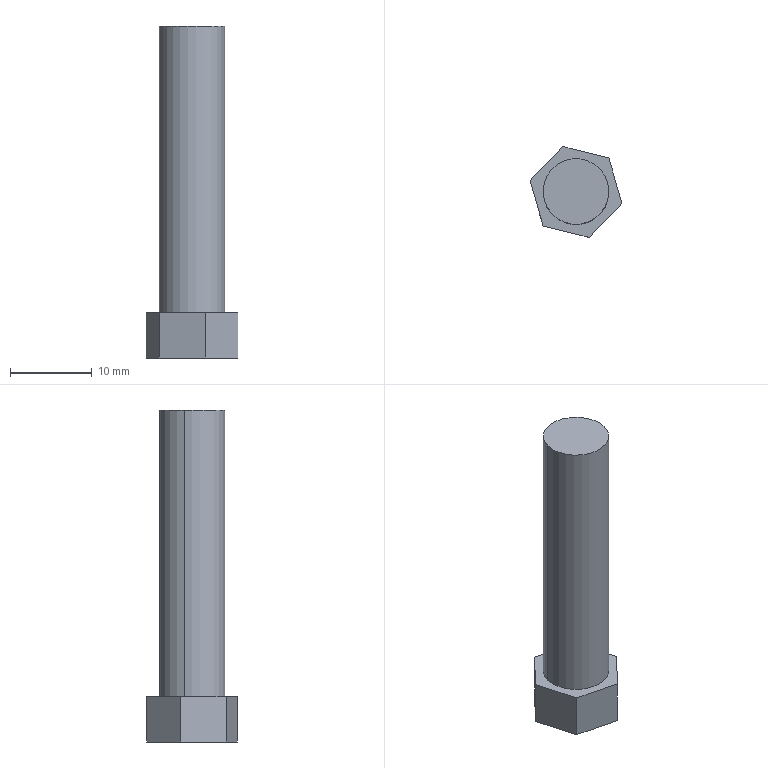Component | SolidWorks | 8Bolt35-1 | 1 solid | 11 faces | box 11.21 x 11.09 x 40.5 mm | volume 2236 mm3 | plane 9 | cylinder 2 | commonest cylinder face diameters 8 x2
STEP:
#1=COLOUR_RGB('',0.7922,0.8196,0.9333);
#2=FILL_AREA_STYLE_COLOUR('',#1);
#3=FILL_AREA_STYLE('',(#2));
#4=SURFACE_STYLE_FILL_AREA(#3);
#5=SURFACE_SIDE_STYLE('',(#4));
#6=SURFACE_STYLE_USAGE(.BOTH.,#5);
#7=PRESENTATION_STYLE_ASSIGNMENT((#6));
#8=CARTESIAN_POINT('',(3.878,5.256,2.511));
#9=VERTEX_POINT('',#8);
#10=CARTESIAN_POINT('',(3.572,5.332,2.511));
#11=VERTEX_POINT('',#10);
#12=CARTESIAN_POINT('',(3.725,5.294,2.511));
#13=DIRECTION('',(0.,0.,1.));
#14=DIRECTION('',(0.9707,-0.2403,0.));
#15=AXIS2_PLACEMENT_3D('',#12,#13,#14);
#16=CIRCLE('',#15,0.1575);
#17=EDGE_CURVE('',#9,#11,#16,.T.);
#18=ORIENTED_EDGE('',*,*,#17,.F.);
#19=CARTESIAN_POINT('',(3.878,5.256,1.133));
#20=VERTEX_POINT('',#19);
#21=CARTESIAN_POINT('',(3.878,5.256,2.511));
#22=DIRECTION('',(0.,0.,-1.));
#23=VECTOR('',#22,39.37);
#24=LINE('',#21,#23);
#25=EDGE_CURVE('',#9,#20,#24,.T.);
#26=ORIENTED_EDGE('',*,*,#25,.T.);
#27=CARTESIAN_POINT('',(3.572,5.332,1.133));
#28=VERTEX_POINT('',#27);
#29=CARTESIAN_POINT('',(3.725,5.294,1.133));
#30=DIRECTION('',(0.,0.,1.));
#31=DIRECTION('',(0.9707,-0.2403,0.));
#32=AXIS2_PLACEMENT_3D('',#29,#30,#31);
#33=CIRCLE('',#32,0.1575);
#34=EDGE_CURVE('',#20,#28,#33,.T.);
#35=ORIENTED_EDGE('',*,*,#34,.T.);
#36=CARTESIAN_POINT('',(3.572,5.332,2.511));
#37=DIRECTION('',(0.,0.,-1.));
#38=VECTOR('',#37,39.37);
#39=LINE('',#36,#38);
#40=EDGE_CURVE('',#11,#28,#39,.T.);
#41=ORIENTED_EDGE('',*,*,#40,.F.);
#42=EDGE_LOOP('',(#18,#26,#35,#41));
#43=FACE_OUTER_BOUND('',#42,.T.);
#44=CARTESIAN_POINT('',(3.725,5.294,2.511));
#45=DIRECTION('',(0.,0.,-1.));
#46=DIRECTION('',(-0.9707,0.2403,0.));
#47=AXIS2_PLACEMENT_3D('',#44,#45,#46);
#48=CYLINDRICAL_SURFACE('',#47,0.1575);
#49=ADVANCED_FACE('',(#43),#48,.T.);
#50=CARTESIAN_POINT('',(3.788,5.075,0.9168));
#51=VERTEX_POINT('',#50);
#52=CARTESIAN_POINT('',(3.946,5.239,0.9168));
#53=VERTEX_POINT('',#52);
#54=CARTESIAN_POINT('',(3.788,5.075,0.9168));
#55=DIRECTION('',(0.6935,0.7205,0.));
#56=VECTOR('',#55,39.37);
#57=LINE('',#54,#56);
#58=EDGE_CURVE('',#51,#53,#57,.T.);
#59=ORIENTED_EDGE('',*,*,#58,.T.);
#60=CARTESIAN_POINT('',(3.946,5.239,1.133));
#61=VERTEX_POINT('',#60);
#62=CARTESIAN_POINT('',(3.946,5.239,1.133));
#63=DIRECTION('',(0.,0.,-1.));
#64=VECTOR('',#63,39.37);
#65=LINE('',#62,#64);
#66=EDGE_CURVE('',#61,#53,#65,.T.);
#67=ORIENTED_EDGE('',*,*,#66,.F.);
#68=CARTESIAN_POINT('',(3.788,5.075,1.133));
#69=VERTEX_POINT('',#68);
#70=CARTESIAN_POINT('',(3.788,5.075,1.133));
#71=DIRECTION('',(0.6935,0.7205,0.));
#72=VECTOR('',#71,39.37);
#73=LINE('',#70,#72);
#74=EDGE_CURVE('',#69,#61,#73,.T.);
#75=ORIENTED_EDGE('',*,*,#74,.F.);
#76=CARTESIAN_POINT('',(3.788,5.075,1.133));
#77=DIRECTION('',(0.,0.,-1.));
#78=VECTOR('',#77,39.37);
#79=LINE('',#76,#78);
#80=EDGE_CURVE('',#69,#51,#79,.T.);
#81=ORIENTED_EDGE('',*,*,#80,.T.);
#82=EDGE_LOOP('',(#59,#67,#75,#81));
#83=FACE_OUTER_BOUND('',#82,.T.);
#84=CARTESIAN_POINT('',(3.788,5.075,1.133));
#85=DIRECTION('',(-0.7205,0.6935,0.));
#86=DIRECTION('',(-0.6935,-0.7205,0.));
#87=AXIS2_PLACEMENT_3D('',#84,#85,#86);
#88=PLANE('',#87);
#89=ADVANCED_FACE('',(#83),#88,.F.);
#90=CARTESIAN_POINT('',(3.883,5.458,0.9168));
#91=VERTEX_POINT('',#90);
#92=CARTESIAN_POINT('',(3.946,5.239,0.9168));
#93=DIRECTION('',(-0.2772,0.9608,0.));
#94=VECTOR('',#93,39.37);
#95=LINE('',#92,#94);
#96=EDGE_CURVE('',#53,#91,#95,.T.);
#97=ORIENTED_EDGE('',*,*,#96,.T.);
#98=CARTESIAN_POINT('',(3.883,5.458,1.133));
#99=VERTEX_POINT('',#98);
#100=CARTESIAN_POINT('',(3.883,5.458,1.133));
#101=DIRECTION('',(0.,0.,-1.));
#102=VECTOR('',#101,39.37);
#103=LINE('',#100,#102);
#104=EDGE_CURVE('',#99,#91,#103,.T.);
#105=ORIENTED_EDGE('',*,*,#104,.F.);
#106=CARTESIAN_POINT('',(3.946,5.239,1.133));
#107=DIRECTION('',(-0.2772,0.9608,0.));
#108=VECTOR('',#107,39.37);
#109=LINE('',#106,#108);
#110=EDGE_CURVE('',#61,#99,#109,.T.);
#111=ORIENTED_EDGE('',*,*,#110,.F.);
#112=ORIENTED_EDGE('',*,*,#66,.T.);
#113=EDGE_LOOP('',(#97,#105,#111,#112));
#114=FACE_OUTER_BOUND('',#113,.T.);
#115=CARTESIAN_POINT('',(3.946,5.239,1.133));
#116=DIRECTION('',(-0.9608,-0.2772,0.));
#117=DIRECTION('',(0.2772,-0.9608,0.));
#118=AXIS2_PLACEMENT_3D('',#115,#116,#117);
#119=PLANE('',#118);
#120=ADVANCED_FACE('',(#114),#119,.F.);
#121=CARTESIAN_POINT('',(3.662,5.512,0.9168));
#122=VERTEX_POINT('',#121);
#123=CARTESIAN_POINT('',(3.883,5.458,0.9168));
#124=DIRECTION('',(-0.9707,0.2403,0.));
#125=VECTOR('',#124,39.37);
#126=LINE('',#123,#125);
#127=EDGE_CURVE('',#91,#122,#126,.T.);
#128=ORIENTED_EDGE('',*,*,#127,.T.);
#129=CARTESIAN_POINT('',(3.662,5.512,1.133));
#130=VERTEX_POINT('',#129);
#131=CARTESIAN_POINT('',(3.662,5.512,1.133));
#132=DIRECTION('',(0.,0.,-1.));
#133=VECTOR('',#132,39.37);
#134=LINE('',#131,#133);
#135=EDGE_CURVE('',#130,#122,#134,.T.);
#136=ORIENTED_EDGE('',*,*,#135,.F.);
#137=CARTESIAN_POINT('',(3.883,5.458,1.133));
#138=DIRECTION('',(-0.9707,0.2403,0.));
#139=VECTOR('',#138,39.37);
#140=LINE('',#137,#139);
#141=EDGE_CURVE('',#99,#130,#140,.T.);
#142=ORIENTED_EDGE('',*,*,#141,.F.);
#143=ORIENTED_EDGE('',*,*,#104,.T.);
#144=EDGE_LOOP('',(#128,#136,#142,#143));
#145=FACE_OUTER_BOUND('',#144,.T.);
#146=CARTESIAN_POINT('',(3.883,5.458,1.133));
#147=DIRECTION('',(-0.2403,-0.9707,0.));
#148=DIRECTION('',(0.,0.,-1.));
#149=AXIS2_PLACEMENT_3D('',#146,#147,#148);
#150=PLANE('',#149);
#151=ADVANCED_FACE('',(#145),#150,.F.);
#152=CARTESIAN_POINT('',(3.504,5.348,0.9168));
#153=VERTEX_POINT('',#152);
#154=CARTESIAN_POINT('',(3.662,5.512,0.9168));
#155=DIRECTION('',(-0.6935,-0.7205,0.));
#156=VECTOR('',#155,39.37);
#157=LINE('',#154,#156);
#158=EDGE_CURVE('',#122,#153,#157,.T.);
#159=ORIENTED_EDGE('',*,*,#158,.T.);
#160=CARTESIAN_POINT('',(3.504,5.348,1.133));
#161=VERTEX_POINT('',#160);
#162=CARTESIAN_POINT('',(3.504,5.348,1.133));
#163=DIRECTION('',(0.,0.,-1.));
#164=VECTOR('',#163,39.37);
#165=LINE('',#162,#164);
#166=EDGE_CURVE('',#161,#153,#165,.T.);
#167=ORIENTED_EDGE('',*,*,#166,.F.);
#168=CARTESIAN_POINT('',(3.662,5.512,1.133));
#169=DIRECTION('',(-0.6935,-0.7205,0.));
#170=VECTOR('',#169,39.37);
#171=LINE('',#168,#170);
#172=EDGE_CURVE('',#130,#161,#171,.T.);
#173=ORIENTED_EDGE('',*,*,#172,.F.);
#174=ORIENTED_EDGE('',*,*,#135,.T.);
#175=EDGE_LOOP('',(#159,#167,#173,#174));
#176=FACE_OUTER_BOUND('',#175,.T.);
#177=CARTESIAN_POINT('',(3.662,5.512,1.133));
#178=DIRECTION('',(0.7205,-0.6935,0.));
#179=DIRECTION('',(0.6935,0.7205,0.));
#180=AXIS2_PLACEMENT_3D('',#177,#178,#179);
#181=PLANE('',#180);
#182=ADVANCED_FACE('',(#176),#181,.F.);
#183=CARTESIAN_POINT('',(3.568,5.13,0.9168));
#184=VERTEX_POINT('',#183);
#185=CARTESIAN_POINT('',(3.504,5.348,0.9168));
#186=DIRECTION('',(0.2772,-0.9608,0.));
#187=VECTOR('',#186,39.37);
#188=LINE('',#185,#187);
#189=EDGE_CURVE('',#153,#184,#188,.T.);
#190=ORIENTED_EDGE('',*,*,#189,.T.);
#191=CARTESIAN_POINT('',(3.568,5.13,1.133));
#192=VERTEX_POINT('',#191);
#193=CARTESIAN_POINT('',(3.568,5.13,1.133));
#194=DIRECTION('',(0.,0.,-1.));
#195=VECTOR('',#194,39.37);
#196=LINE('',#193,#195);
#197=EDGE_CURVE('',#192,#184,#196,.T.);
#198=ORIENTED_EDGE('',*,*,#197,.F.);
#199=CARTESIAN_POINT('',(3.504,5.348,1.133));
#200=DIRECTION('',(0.2772,-0.9608,0.));
#201=VECTOR('',#200,39.37);
#202=LINE('',#199,#201);
#203=EDGE_CURVE('',#161,#192,#202,.T.);
#204=ORIENTED_EDGE('',*,*,#203,.F.);
#205=ORIENTED_EDGE('',*,*,#166,.T.);
#206=EDGE_LOOP('',(#190,#198,#204,#205));
#207=FACE_OUTER_BOUND('',#206,.T.);
#208=CARTESIAN_POINT('',(3.504,5.348,1.133));
#209=DIRECTION('',(0.9608,0.2772,0.));
#210=DIRECTION('',(-0.2772,0.9608,0.));
#211=AXIS2_PLACEMENT_3D('',#208,#209,#210);
#212=PLANE('',#211);
#213=ADVANCED_FACE('',(#207),#212,.F.);
#214=CARTESIAN_POINT('',(3.568,5.13,0.9168));
#215=DIRECTION('',(0.9707,-0.2403,0.));
#216=VECTOR('',#215,39.37);
#217=LINE('',#214,#216);
#218=EDGE_CURVE('',#184,#51,#217,.T.);
#219=ORIENTED_EDGE('',*,*,#218,.T.);
#220=ORIENTED_EDGE('',*,*,#80,.F.);
#221=CARTESIAN_POINT('',(3.568,5.13,1.133));
#222=DIRECTION('',(0.9707,-0.2403,0.));
#223=VECTOR('',#222,39.37);
#224=LINE('',#221,#223);
#225=EDGE_CURVE('',#192,#69,#224,.T.);
#226=ORIENTED_EDGE('',*,*,#225,.F.);
#227=ORIENTED_EDGE('',*,*,#197,.T.);
#228=EDGE_LOOP('',(#219,#220,#226,#227));
#229=FACE_OUTER_BOUND('',#228,.T.);
#230=CARTESIAN_POINT('',(3.568,5.13,1.133));
#231=DIRECTION('',(0.2403,0.9707,0.));
#232=DIRECTION('',(-0.9707,0.2403,0.));
#233=AXIS2_PLACEMENT_3D('',#230,#231,#232);
#234=PLANE('',#233);
#235=ADVANCED_FACE('',(#229),#234,.F.);
#236=CARTESIAN_POINT('',(3.725,5.294,1.133));
#237=DIRECTION('',(0.,0.,1.));
#238=DIRECTION('',(0.9707,-0.2403,0.));
#239=AXIS2_PLACEMENT_3D('',#236,#237,#238);
#240=CIRCLE('',#239,0.1575);
#241=EDGE_CURVE('',#28,#20,#240,.T.);
#242=ORIENTED_EDGE('',*,*,#241,.F.);
#243=ORIENTED_EDGE('',*,*,#34,.F.);
#244=EDGE_LOOP('',(#242,#243));
#245=FACE_BOUND('',#244,.T.);
#246=ORIENTED_EDGE('',*,*,#74,.T.);
#247=ORIENTED_EDGE('',*,*,#110,.T.);
#248=ORIENTED_EDGE('',*,*,#141,.T.);
#249=ORIENTED_EDGE('',*,*,#172,.T.);
#250=ORIENTED_EDGE('',*,*,#203,.T.);
#251=ORIENTED_EDGE('',*,*,#225,.T.);
#252=EDGE_LOOP('',(#246,#247,#248,#249,#250,#251));
#253=FACE_OUTER_BOUND('',#252,.T.);
#254=CARTESIAN_POINT('',(3.725,5.294,1.133));
#255=DIRECTION('',(0.,0.,1.));
#256=DIRECTION('',(0.9707,-0.2403,0.));
#257=AXIS2_PLACEMENT_3D('',#254,#255,#256);
#258=PLANE('',#257);
#259=ADVANCED_FACE('',(#245,#253),#258,.T.);
#260=ORIENTED_EDGE('',*,*,#58,.F.);
#261=ORIENTED_EDGE('',*,*,#218,.F.);
#262=ORIENTED_EDGE('',*,*,#189,.F.);
#263=ORIENTED_EDGE('',*,*,#158,.F.);
#264=ORIENTED_EDGE('',*,*,#127,.F.);
#265=ORIENTED_EDGE('',*,*,#96,.F.);
#266=EDGE_LOOP('',(#260,#261,#262,#263,#264,#265));
#267=FACE_OUTER_BOUND('',#266,.T.);
#268=CARTESIAN_POINT('',(3.725,5.294,0.9168));
#269=DIRECTION('',(0.,0.,1.));
#270=DIRECTION('',(0.9707,-0.2403,0.));
#271=AXIS2_PLACEMENT_3D('',#268,#269,#270);
#272=PLANE('',#271);
#273=ADVANCED_FACE('',(#267),#272,.F.);
#274=ORIENTED_EDGE('',*,*,#25,.F.);
#275=CARTESIAN_POINT('',(3.725,5.294,2.511));
#276=DIRECTION('',(0.,0.,1.));
#277=DIRECTION('',(0.9707,-0.2403,0.));
#278=AXIS2_PLACEMENT_3D('',#275,#276,#277);
#279=CIRCLE('',#278,0.1575);
#280=EDGE_CURVE('',#11,#9,#279,.T.);
#281=ORIENTED_EDGE('',*,*,#280,.F.);
#282=ORIENTED_EDGE('',*,*,#40,.T.);
#283=ORIENTED_EDGE('',*,*,#241,.T.);
#284=EDGE_LOOP('',(#274,#281,#282,#283));
#285=FACE_OUTER_BOUND('',#284,.T.);
#286=CARTESIAN_POINT('',(3.725,5.294,2.511));
#287=DIRECTION('',(0.,0.,-1.));
#288=DIRECTION('',(-0.9707,0.2403,0.));
#289=AXIS2_PLACEMENT_3D('',#286,#287,#288);
#290=CYLINDRICAL_SURFACE('',#289,0.1575);
#291=ADVANCED_FACE('',(#285),#290,.T.);
#292=ORIENTED_EDGE('',*,*,#280,.T.);
#293=ORIENTED_EDGE('',*,*,#17,.T.);
#294=EDGE_LOOP('',(#292,#293));
#295=FACE_OUTER_BOUND('',#294,.T.);
#296=CARTESIAN_POINT('',(3.725,5.294,2.511));
#297=DIRECTION('',(0.,0.,1.));
#298=DIRECTION('',(0.9707,-0.2403,0.));
#299=AXIS2_PLACEMENT_3D('',#296,#297,#298);
#300=PLANE('',#299);
#301=ADVANCED_FACE('',(#295),#300,.T.);
#302=CLOSED_SHELL('',(#49,#89,#120,#151,#182,#213,#235,#259,#273,#291,#301));
#303=MANIFOLD_SOLID_BREP('',#302);
#304=STYLED_ITEM('',(#7),#303);
#305=(LENGTH_UNIT()NAMED_UNIT(*)SI_UNIT($,.METRE.));
#306=LENGTH_MEASURE_WITH_UNIT(LENGTH_MEASURE(0.0254),#305);
#307=DIMENSIONAL_EXPONENTS(1.,0.,0.,0.,0.,0.,0.);
#308=(CONVERSION_BASED_UNIT('',#306)LENGTH_UNIT()NAMED_UNIT(#307));
#309=UNCERTAINTY_MEASURE_WITH_UNIT(LENGTH_MEASURE(0.00001),#308,'','');
#310=(NAMED_UNIT(*)PLANE_ANGLE_UNIT()SI_UNIT($,.RADIAN.));
#311=(NAMED_UNIT(*)SI_UNIT($,.STERADIAN.)SOLID_ANGLE_UNIT());
#312=(GEOMETRIC_REPRESENTATION_CONTEXT(3)GLOBAL_UNCERTAINTY_ASSIGNED_CONTEXT((#309))GLOBAL_UNIT_ASSIGNED_CONTEXT((#308,#310,#311))REPRESENTATION_CONTEXT('',''));
#313=MECHANICAL_DESIGN_GEOMETRIC_PRESENTATION_REPRESENTATION('',(#304),#312);
#314=CARTESIAN_POINT('',(0.,0.,0.));
#315=DIRECTION('',(0.,0.,1.));
#316=DIRECTION('',(1.,0.,0.));
#317=AXIS2_PLACEMENT_3D('',#314,#315,#316);
#318=(LENGTH_UNIT()NAMED_UNIT(*)SI_UNIT($,.METRE.));
#319=LENGTH_MEASURE_WITH_UNIT(LENGTH_MEASURE(0.0254),#318);
#320=DIMENSIONAL_EXPONENTS(1.,0.,0.,0.,0.,0.,0.);
#321=(CONVERSION_BASED_UNIT('',#319)LENGTH_UNIT()NAMED_UNIT(#320));
#322=UNCERTAINTY_MEASURE_WITH_UNIT(LENGTH_MEASURE(0.00001),#321,'','');
#323=(NAMED_UNIT(*)PLANE_ANGLE_UNIT()SI_UNIT($,.RADIAN.));
#324=(NAMED_UNIT(*)SI_UNIT($,.STERADIAN.)SOLID_ANGLE_UNIT());
#325=(GEOMETRIC_REPRESENTATION_CONTEXT(3)GLOBAL_UNCERTAINTY_ASSIGNED_CONTEXT((#322))GLOBAL_UNIT_ASSIGNED_CONTEXT((#321,#323,#324))REPRESENTATION_CONTEXT('',''));
#326=ADVANCED_BREP_SHAPE_REPRESENTATION('',(#303,#317),#325);
#327=PRESENTATION_LAYER_ASSIGNMENT('','',(#304));